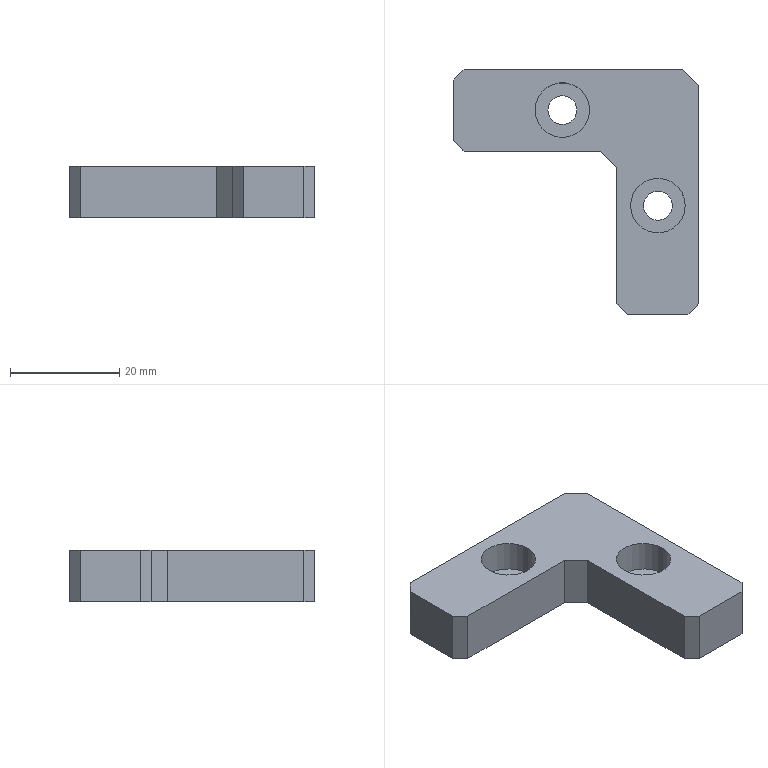Component | SolidWorks | --MA18S20041AxisStopBlock1-1 | 1 solid | 24 faces | box 45 x 45 x 9.5 mm | volume 9548 mm3 | plane 16 | cylinder 8 | commonest cylinder face diameters 10 x4 5.3 x4
build123d program:
from build123d import *

# Parameters (mm, degrees)
EXTRUDE_THIN1_DEPTH                                  = 9.5
CHAMFER1_SIZE                                        = 3
CHAMFER2_SIZE                                        = 2
HOLE_SIZE_ACCORDING_TO_THE_TYPE_OF_HEXAG_D           = 5.3
HOLE_SIZE_ACCORDING_TO_THE_TYPE_OF_HEXAG_CBORE_D     = 10
HOLE_SIZE_ACCORDING_TO_THE_TYPE_OF_HEXAG_CBORE_DEPTH = 5.7


with BuildPart() as part:
    # Sketch1 → Extrude-Thin1 (new body)
    with BuildSketch(Plane.XY):
        Polygon((0, 0), (45, 0), (45, -45), (30, -45), (30, -15), (0, -15), align=None)
    extrude(amount=EXTRUDE_THIN1_DEPTH)

    # Chamfer1
    chamfer1_edges = [part.edges().sort_by_distance(p)[0] for p in [
        (30, -15, 4.75),
        (45, 0, 4.75),
    ]]
    chamfer(chamfer1_edges, length=CHAMFER1_SIZE)

    # Chamfer2
    chamfer2_edges = [part.edges().sort_by_distance(p)[0] for p in [
        (0, -15, 4.75),
        (0, 0, 4.75),
        (45, -45, 4.75),
        (30, -45, 4.75),
    ]]
    chamfer(chamfer2_edges, length=CHAMFER2_SIZE)

    # Hole Size according to the type of Hexag (through all)
    with Locations(Plane.XY.offset(9.5)):
        with Locations((37.5, -25), (20, -7.5)):
            CounterBoreHole(HOLE_SIZE_ACCORDING_TO_THE_TYPE_OF_HEXAG_D / 2, HOLE_SIZE_ACCORDING_TO_THE_TYPE_OF_HEXAG_CBORE_D / 2, HOLE_SIZE_ACCORDING_TO_THE_TYPE_OF_HEXAG_CBORE_DEPTH)


solid = part.part

# Placed as in the assembly
solid = solid.moved(Location((-175.456, 104.199, 68), (0, 0, 0)))
STEP:
#1=COLOUR_RGB('',0.7922,0.8196,0.9333);
#2=FILL_AREA_STYLE_COLOUR('',#1);
#3=FILL_AREA_STYLE('',(#2));
#4=SURFACE_STYLE_FILL_AREA(#3);
#5=SURFACE_SIDE_STYLE('',(#4));
#6=SURFACE_STYLE_USAGE(.BOTH.,#5);
#7=PRESENTATION_STYLE_ASSIGNMENT((#6));
#8=CARTESIAN_POINT('',(-5.628,3.118,2.827));
#9=VERTEX_POINT('',#8);
#10=CARTESIAN_POINT('',(-5.234,3.118,2.827));
#11=VERTEX_POINT('',#10);
#12=CARTESIAN_POINT('',(-5.431,3.118,2.827));
#13=DIRECTION('',(0.,0.,1.));
#14=DIRECTION('',(1.,0.,0.));
#15=AXIS2_PLACEMENT_3D('',#12,#13,#14);
#16=CIRCLE('',#15,0.1969);
#17=EDGE_CURVE('',#9,#11,#16,.T.);
#18=ORIENTED_EDGE('',*,*,#17,.F.);
#19=CARTESIAN_POINT('',(-5.628,3.118,3.051));
#20=VERTEX_POINT('',#19);
#21=CARTESIAN_POINT('',(-5.628,3.118,3.051));
#22=DIRECTION('',(0.,0.,1.));
#23=VECTOR('',#22,39.37);
#24=LINE('',#21,#23);
#25=EDGE_CURVE('',#9,#20,#24,.T.);
#26=ORIENTED_EDGE('',*,*,#25,.T.);
#27=CARTESIAN_POINT('',(-5.234,3.118,3.051));
#28=VERTEX_POINT('',#27);
#29=CARTESIAN_POINT('',(-5.431,3.118,3.051));
#30=DIRECTION('',(0.,0.,1.));
#31=DIRECTION('',(1.,0.,0.));
#32=AXIS2_PLACEMENT_3D('',#29,#30,#31);
#33=CIRCLE('',#32,0.1969);
#34=EDGE_CURVE('',#20,#28,#33,.T.);
#35=ORIENTED_EDGE('',*,*,#34,.T.);
#36=CARTESIAN_POINT('',(-5.234,3.118,3.051));
#37=DIRECTION('',(0.,0.,1.));
#38=VECTOR('',#37,39.37);
#39=LINE('',#36,#38);
#40=EDGE_CURVE('',#11,#28,#39,.T.);
#41=ORIENTED_EDGE('',*,*,#40,.F.);
#42=EDGE_LOOP('',(#18,#26,#35,#41));
#43=FACE_OUTER_BOUND('',#42,.T.);
#44=CARTESIAN_POINT('',(-5.431,3.118,3.051));
#45=DIRECTION('',(0.,0.,1.));
#46=DIRECTION('',(1.,0.,0.));
#47=AXIS2_PLACEMENT_3D('',#44,#45,#46);
#48=CYLINDRICAL_SURFACE('',#47,0.1969);
#49=ADVANCED_FACE('',(#43),#48,.F.);
#50=CARTESIAN_POINT('',(-5.536,3.118,2.677));
#51=VERTEX_POINT('',#50);
#52=CARTESIAN_POINT('',(-5.327,3.118,2.677));
#53=VERTEX_POINT('',#52);
#54=CARTESIAN_POINT('',(-5.431,3.118,2.677));
#55=DIRECTION('',(0.,0.,1.));
#56=DIRECTION('',(1.,0.,0.));
#57=AXIS2_PLACEMENT_3D('',#54,#55,#56);
#58=CIRCLE('',#57,0.1043);
#59=EDGE_CURVE('',#51,#53,#58,.T.);
#60=ORIENTED_EDGE('',*,*,#59,.F.);
#61=CARTESIAN_POINT('',(-5.536,3.118,2.827));
#62=VERTEX_POINT('',#61);
#63=CARTESIAN_POINT('',(-5.536,3.118,3.051));
#64=DIRECTION('',(0.,0.,1.));
#65=VECTOR('',#64,39.37);
#66=LINE('',#63,#65);
#67=EDGE_CURVE('',#51,#62,#66,.T.);
#68=ORIENTED_EDGE('',*,*,#67,.T.);
#69=CARTESIAN_POINT('',(-5.327,3.118,2.827));
#70=VERTEX_POINT('',#69);
#71=CARTESIAN_POINT('',(-5.431,3.118,2.827));
#72=DIRECTION('',(0.,0.,1.));
#73=DIRECTION('',(1.,0.,0.));
#74=AXIS2_PLACEMENT_3D('',#71,#72,#73);
#75=CIRCLE('',#74,0.1043);
#76=EDGE_CURVE('',#62,#70,#75,.T.);
#77=ORIENTED_EDGE('',*,*,#76,.T.);
#78=CARTESIAN_POINT('',(-5.327,3.118,3.051));
#79=DIRECTION('',(0.,0.,1.));
#80=VECTOR('',#79,39.37);
#81=LINE('',#78,#80);
#82=EDGE_CURVE('',#53,#70,#81,.T.);
#83=ORIENTED_EDGE('',*,*,#82,.F.);
#84=EDGE_LOOP('',(#60,#68,#77,#83));
#85=FACE_OUTER_BOUND('',#84,.T.);
#86=CARTESIAN_POINT('',(-5.431,3.118,3.051));
#87=DIRECTION('',(0.,0.,1.));
#88=DIRECTION('',(1.,0.,0.));
#89=AXIS2_PLACEMENT_3D('',#86,#87,#88);
#90=CYLINDRICAL_SURFACE('',#89,0.1043);
#91=ADVANCED_FACE('',(#85),#90,.F.);
#92=CARTESIAN_POINT('',(-6.317,3.807,2.827));
#93=VERTEX_POINT('',#92);
#94=CARTESIAN_POINT('',(-5.923,3.807,2.827));
#95=VERTEX_POINT('',#94);
#96=CARTESIAN_POINT('',(-6.12,3.807,2.827));
#97=DIRECTION('',(0.,0.,1.));
#98=DIRECTION('',(1.,0.,0.));
#99=AXIS2_PLACEMENT_3D('',#96,#97,#98);
#100=CIRCLE('',#99,0.1969);
#101=EDGE_CURVE('',#93,#95,#100,.T.);
#102=ORIENTED_EDGE('',*,*,#101,.F.);
#103=CARTESIAN_POINT('',(-6.317,3.807,3.051));
#104=VERTEX_POINT('',#103);
#105=CARTESIAN_POINT('',(-6.317,3.807,3.051));
#106=DIRECTION('',(0.,0.,1.));
#107=VECTOR('',#106,39.37);
#108=LINE('',#105,#107);
#109=EDGE_CURVE('',#93,#104,#108,.T.);
#110=ORIENTED_EDGE('',*,*,#109,.T.);
#111=CARTESIAN_POINT('',(-5.923,3.807,3.051));
#112=VERTEX_POINT('',#111);
#113=CARTESIAN_POINT('',(-6.12,3.807,3.051));
#114=DIRECTION('',(0.,0.,1.));
#115=DIRECTION('',(1.,0.,0.));
#116=AXIS2_PLACEMENT_3D('',#113,#114,#115);
#117=CIRCLE('',#116,0.1969);
#118=EDGE_CURVE('',#104,#112,#117,.T.);
#119=ORIENTED_EDGE('',*,*,#118,.T.);
#120=CARTESIAN_POINT('',(-5.923,3.807,3.051));
#121=DIRECTION('',(0.,0.,1.));
#122=VECTOR('',#121,39.37);
#123=LINE('',#120,#122);
#124=EDGE_CURVE('',#95,#112,#123,.T.);
#125=ORIENTED_EDGE('',*,*,#124,.F.);
#126=EDGE_LOOP('',(#102,#110,#119,#125));
#127=FACE_OUTER_BOUND('',#126,.T.);
#128=CARTESIAN_POINT('',(-6.12,3.807,3.051));
#129=DIRECTION('',(0.,0.,1.));
#130=DIRECTION('',(1.,0.,0.));
#131=AXIS2_PLACEMENT_3D('',#128,#129,#130);
#132=CYLINDRICAL_SURFACE('',#131,0.1969);
#133=ADVANCED_FACE('',(#127),#132,.F.);
#134=CARTESIAN_POINT('',(-6.225,3.807,2.677));
#135=VERTEX_POINT('',#134);
#136=CARTESIAN_POINT('',(-6.016,3.807,2.677));
#137=VERTEX_POINT('',#136);
#138=CARTESIAN_POINT('',(-6.12,3.807,2.677));
#139=DIRECTION('',(0.,0.,1.));
#140=DIRECTION('',(1.,0.,0.));
#141=AXIS2_PLACEMENT_3D('',#138,#139,#140);
#142=CIRCLE('',#141,0.1043);
#143=EDGE_CURVE('',#135,#137,#142,.T.);
#144=ORIENTED_EDGE('',*,*,#143,.F.);
#145=CARTESIAN_POINT('',(-6.225,3.807,2.827));
#146=VERTEX_POINT('',#145);
#147=CARTESIAN_POINT('',(-6.225,3.807,3.051));
#148=DIRECTION('',(0.,0.,1.));
#149=VECTOR('',#148,39.37);
#150=LINE('',#147,#149);
#151=EDGE_CURVE('',#135,#146,#150,.T.);
#152=ORIENTED_EDGE('',*,*,#151,.T.);
#153=CARTESIAN_POINT('',(-6.016,3.807,2.827));
#154=VERTEX_POINT('',#153);
#155=CARTESIAN_POINT('',(-6.12,3.807,2.827));
#156=DIRECTION('',(0.,0.,1.));
#157=DIRECTION('',(1.,0.,0.));
#158=AXIS2_PLACEMENT_3D('',#155,#156,#157);
#159=CIRCLE('',#158,0.1043);
#160=EDGE_CURVE('',#146,#154,#159,.T.);
#161=ORIENTED_EDGE('',*,*,#160,.T.);
#162=CARTESIAN_POINT('',(-6.016,3.807,3.051));
#163=DIRECTION('',(0.,0.,1.));
#164=VECTOR('',#163,39.37);
#165=LINE('',#162,#164);
#166=EDGE_CURVE('',#137,#154,#165,.T.);
#167=ORIENTED_EDGE('',*,*,#166,.F.);
#168=EDGE_LOOP('',(#144,#152,#161,#167));
#169=FACE_OUTER_BOUND('',#168,.T.);
#170=CARTESIAN_POINT('',(-6.12,3.807,3.051));
#171=DIRECTION('',(0.,0.,1.));
#172=DIRECTION('',(1.,0.,0.));
#173=AXIS2_PLACEMENT_3D('',#170,#171,#172);
#174=CYLINDRICAL_SURFACE('',#173,0.1043);
#175=ADVANCED_FACE('',(#169),#174,.F.);
#176=CARTESIAN_POINT('',(-5.431,3.118,3.051));
#177=DIRECTION('',(0.,0.,1.));
#178=DIRECTION('',(1.,0.,0.));
#179=AXIS2_PLACEMENT_3D('',#176,#177,#178);
#180=CIRCLE('',#179,0.1969);
#181=EDGE_CURVE('',#28,#20,#180,.T.);
#182=ORIENTED_EDGE('',*,*,#181,.F.);
#183=ORIENTED_EDGE('',*,*,#34,.F.);
#184=EDGE_LOOP('',(#182,#183));
#185=FACE_BOUND('',#184,.T.);
#186=CARTESIAN_POINT('',(-5.215,2.331,3.051));
#187=VERTEX_POINT('',#186);
#188=CARTESIAN_POINT('',(-5.648,2.331,3.051));
#189=VERTEX_POINT('',#188);
#190=CARTESIAN_POINT('',(-5.136,2.331,3.051));
#191=DIRECTION('',(-1.,0.,0.));
#192=VECTOR('',#191,39.37);
#193=LINE('',#190,#192);
#194=EDGE_CURVE('',#187,#189,#193,.T.);
#195=ORIENTED_EDGE('',*,*,#194,.F.);
#196=CARTESIAN_POINT('',(-5.136,2.409,3.051));
#197=VERTEX_POINT('',#196);
#198=CARTESIAN_POINT('',(-5.136,2.409,3.051));
#199=DIRECTION('',(0.7071,0.7071,0.));
#200=VECTOR('',#199,39.37);
#201=LINE('',#198,#200);
#202=EDGE_CURVE('',#187,#197,#201,.T.);
#203=ORIENTED_EDGE('',*,*,#202,.T.);
#204=CARTESIAN_POINT('',(-5.136,3.984,3.051));
#205=VERTEX_POINT('',#204);
#206=CARTESIAN_POINT('',(-5.136,4.102,3.051));
#207=DIRECTION('',(0.,-1.,0.));
#208=VECTOR('',#207,39.37);
#209=LINE('',#206,#208);
#210=EDGE_CURVE('',#205,#197,#209,.T.);
#211=ORIENTED_EDGE('',*,*,#210,.F.);
#212=CARTESIAN_POINT('',(-5.254,4.102,3.051));
#213=VERTEX_POINT('',#212);
#214=CARTESIAN_POINT('',(-5.254,4.102,3.051));
#215=DIRECTION('',(-0.7071,0.7071,0.));
#216=VECTOR('',#215,39.37);
#217=LINE('',#214,#216);
#218=EDGE_CURVE('',#205,#213,#217,.T.);
#219=ORIENTED_EDGE('',*,*,#218,.T.);
#220=CARTESIAN_POINT('',(-6.829,4.102,3.051));
#221=VERTEX_POINT('',#220);
#222=CARTESIAN_POINT('',(-6.908,4.102,3.051));
#223=DIRECTION('',(1.,0.,0.));
#224=VECTOR('',#223,39.37);
#225=LINE('',#222,#224);
#226=EDGE_CURVE('',#221,#213,#225,.T.);
#227=ORIENTED_EDGE('',*,*,#226,.F.);
#228=CARTESIAN_POINT('',(-6.908,4.024,3.051));
#229=VERTEX_POINT('',#228);
#230=CARTESIAN_POINT('',(-6.908,4.024,3.051));
#231=DIRECTION('',(-0.7071,-0.7071,0.));
#232=VECTOR('',#231,39.37);
#233=LINE('',#230,#232);
#234=EDGE_CURVE('',#221,#229,#233,.T.);
#235=ORIENTED_EDGE('',*,*,#234,.T.);
#236=CARTESIAN_POINT('',(-6.908,3.591,3.051));
#237=VERTEX_POINT('',#236);
#238=CARTESIAN_POINT('',(-6.908,3.512,3.051));
#239=DIRECTION('',(0.,1.,0.));
#240=VECTOR('',#239,39.37);
#241=LINE('',#238,#240);
#242=EDGE_CURVE('',#237,#229,#241,.T.);
#243=ORIENTED_EDGE('',*,*,#242,.F.);
#244=CARTESIAN_POINT('',(-6.829,3.512,3.051));
#245=VERTEX_POINT('',#244);
#246=CARTESIAN_POINT('',(-6.829,3.512,3.051));
#247=DIRECTION('',(0.7071,-0.7071,0.));
#248=VECTOR('',#247,39.37);
#249=LINE('',#246,#248);
#250=EDGE_CURVE('',#237,#245,#249,.T.);
#251=ORIENTED_EDGE('',*,*,#250,.T.);
#252=CARTESIAN_POINT('',(-5.845,3.512,3.051));
#253=VERTEX_POINT('',#252);
#254=CARTESIAN_POINT('',(-6.908,3.512,3.051));
#255=DIRECTION('',(1.,0.,0.));
#256=VECTOR('',#255,39.37);
#257=LINE('',#254,#256);
#258=EDGE_CURVE('',#245,#253,#257,.T.);
#259=ORIENTED_EDGE('',*,*,#258,.T.);
#260=CARTESIAN_POINT('',(-5.727,3.394,3.051));
#261=VERTEX_POINT('',#260);
#262=CARTESIAN_POINT('',(-5.195,2.862,3.051));
#263=DIRECTION('',(0.7071,-0.7071,0.));
#264=VECTOR('',#263,39.37);
#265=LINE('',#262,#264);
#266=EDGE_CURVE('',#253,#261,#265,.T.);
#267=ORIENTED_EDGE('',*,*,#266,.T.);
#268=CARTESIAN_POINT('',(-5.727,2.409,3.051));
#269=VERTEX_POINT('',#268);
#270=CARTESIAN_POINT('',(-5.727,4.102,3.051));
#271=DIRECTION('',(0.,-1.,0.));
#272=VECTOR('',#271,39.37);
#273=LINE('',#270,#272);
#274=EDGE_CURVE('',#261,#269,#273,.T.);
#275=ORIENTED_EDGE('',*,*,#274,.T.);
#276=CARTESIAN_POINT('',(-5.648,2.331,3.051));
#277=DIRECTION('',(0.7071,-0.7071,0.));
#278=VECTOR('',#277,39.37);
#279=LINE('',#276,#278);
#280=EDGE_CURVE('',#269,#189,#279,.T.);
#281=ORIENTED_EDGE('',*,*,#280,.T.);
#282=EDGE_LOOP('',(#195,#203,#211,#219,#227,#235,#243,#251,#259,#267,#275,#281));
#283=FACE_OUTER_BOUND('',#282,.T.);
#284=CARTESIAN_POINT('',(-6.12,3.807,3.051));
#285=DIRECTION('',(0.,0.,1.));
#286=DIRECTION('',(1.,0.,0.));
#287=AXIS2_PLACEMENT_3D('',#284,#285,#286);
#288=CIRCLE('',#287,0.1969);
#289=EDGE_CURVE('',#112,#104,#288,.T.);
#290=ORIENTED_EDGE('',*,*,#289,.F.);
#291=ORIENTED_EDGE('',*,*,#118,.F.);
#292=EDGE_LOOP('',(#290,#291));
#293=FACE_BOUND('',#292,.T.);
#294=CARTESIAN_POINT('',(-5.727,2.331,3.051));
#295=DIRECTION('',(0.,0.,-1.));
#296=DIRECTION('',(-1.,0.,0.));
#297=AXIS2_PLACEMENT_3D('',#294,#295,#296);
#298=PLANE('',#297);
#299=ADVANCED_FACE('',(#185,#283,#293),#298,.F.);
#300=CARTESIAN_POINT('',(-5.727,3.394,2.677));
#301=VERTEX_POINT('',#300);
#302=CARTESIAN_POINT('',(-5.727,2.409,2.677));
#303=VERTEX_POINT('',#302);
#304=CARTESIAN_POINT('',(-5.727,4.102,2.677));
#305=DIRECTION('',(0.,-1.,0.));
#306=VECTOR('',#305,39.37);
#307=LINE('',#304,#306);
#308=EDGE_CURVE('',#301,#303,#307,.T.);
#309=ORIENTED_EDGE('',*,*,#308,.T.);
#310=CARTESIAN_POINT('',(-5.727,2.409,3.051));
#311=DIRECTION('',(0.,0.,1.));
#312=VECTOR('',#311,39.37);
#313=LINE('',#310,#312);
#314=EDGE_CURVE('',#303,#269,#313,.T.);
#315=ORIENTED_EDGE('',*,*,#314,.T.);
#316=ORIENTED_EDGE('',*,*,#274,.F.);
#317=CARTESIAN_POINT('',(-5.727,3.394,2.677));
#318=DIRECTION('',(0.,0.,-1.));
#319=VECTOR('',#318,39.37);
#320=LINE('',#317,#319);
#321=EDGE_CURVE('',#261,#301,#320,.T.);
#322=ORIENTED_EDGE('',*,*,#321,.T.);
#323=EDGE_LOOP('',(#309,#315,#316,#322));
#324=FACE_OUTER_BOUND('',#323,.T.);
#325=CARTESIAN_POINT('',(-5.727,4.102,3.051));
#326=DIRECTION('',(1.,0.,0.));
#327=DIRECTION('',(-0.,1.,0.));
#328=AXIS2_PLACEMENT_3D('',#325,#326,#327);
#329=PLANE('',#328);
#330=ADVANCED_FACE('',(#324),#329,.F.);
#331=CARTESIAN_POINT('',(-5.215,2.331,2.677));
#332=VERTEX_POINT('',#331);
#333=CARTESIAN_POINT('',(-5.648,2.331,2.677));
#334=VERTEX_POINT('',#333);
#335=CARTESIAN_POINT('',(-5.136,2.331,2.677));
#336=DIRECTION('',(-1.,0.,0.));
#337=VECTOR('',#336,39.37);
#338=LINE('',#335,#337);
#339=EDGE_CURVE('',#332,#334,#338,.T.);
#340=ORIENTED_EDGE('',*,*,#339,.F.);
#341=CARTESIAN_POINT('',(-5.215,2.331,3.051));
#342=DIRECTION('',(0.,0.,1.));
#343=VECTOR('',#342,39.37);
#344=LINE('',#341,#343);
#345=EDGE_CURVE('',#332,#187,#344,.T.);
#346=ORIENTED_EDGE('',*,*,#345,.T.);
#347=ORIENTED_EDGE('',*,*,#194,.T.);
#348=CARTESIAN_POINT('',(-5.648,2.331,2.677));
#349=DIRECTION('',(0.,0.,-1.));
#350=VECTOR('',#349,39.37);
#351=LINE('',#348,#350);
#352=EDGE_CURVE('',#189,#334,#351,.T.);
#353=ORIENTED_EDGE('',*,*,#352,.T.);
#354=EDGE_LOOP('',(#340,#346,#347,#353));
#355=FACE_OUTER_BOUND('',#354,.T.);
#356=CARTESIAN_POINT('',(-5.136,2.331,3.051));
#357=DIRECTION('',(0.,-1.,0.));
#358=DIRECTION('',(0.,0.,-1.));
#359=AXIS2_PLACEMENT_3D('',#356,#357,#358);
#360=PLANE('',#359);
#361=ADVANCED_FACE('',(#355),#360,.T.);
#362=ORIENTED_EDGE('',*,*,#210,.T.);
#363=CARTESIAN_POINT('',(-5.136,2.409,2.677));
#364=VERTEX_POINT('',#363);
#365=CARTESIAN_POINT('',(-5.136,2.409,3.051));
#366=DIRECTION('',(0.,0.,-1.));
#367=VECTOR('',#366,39.37);
#368=LINE('',#365,#367);
#369=EDGE_CURVE('',#197,#364,#368,.T.);
#370=ORIENTED_EDGE('',*,*,#369,.T.);
#371=CARTESIAN_POINT('',(-5.136,3.984,2.677));
#372=VERTEX_POINT('',#371);
#373=CARTESIAN_POINT('',(-5.136,4.102,2.677));
#374=DIRECTION('',(0.,-1.,0.));
#375=VECTOR('',#374,39.37);
#376=LINE('',#373,#375);
#377=EDGE_CURVE('',#372,#364,#376,.T.);
#378=ORIENTED_EDGE('',*,*,#377,.F.);
#379=CARTESIAN_POINT('',(-5.136,3.984,3.051));
#380=DIRECTION('',(0.,0.,1.));
#381=VECTOR('',#380,39.37);
#382=LINE('',#379,#381);
#383=EDGE_CURVE('',#372,#205,#382,.T.);
#384=ORIENTED_EDGE('',*,*,#383,.T.);
#385=EDGE_LOOP('',(#362,#370,#378,#384));
#386=FACE_OUTER_BOUND('',#385,.T.);
#387=CARTESIAN_POINT('',(-5.136,4.102,3.051));
#388=DIRECTION('',(1.,0.,0.));
#389=DIRECTION('',(-0.,1.,0.));
#390=AXIS2_PLACEMENT_3D('',#387,#388,#389);
#391=PLANE('',#390);
#392=ADVANCED_FACE('',(#386),#391,.T.);
#393=CARTESIAN_POINT('',(-6.829,4.102,2.677));
#394=VERTEX_POINT('',#393);
#395=CARTESIAN_POINT('',(-5.254,4.102,2.677));
#396=VERTEX_POINT('',#395);
#397=CARTESIAN_POINT('',(-6.908,4.102,2.677));
#398=DIRECTION('',(1.,0.,0.));
#399=VECTOR('',#398,39.37);
#400=LINE('',#397,#399);
#401=EDGE_CURVE('',#394,#396,#400,.T.);
#402=ORIENTED_EDGE('',*,*,#401,.F.);
#403=CARTESIAN_POINT('',(-6.829,4.102,3.051));
#404=DIRECTION('',(0.,0.,1.));
#405=VECTOR('',#404,39.37);
#406=LINE('',#403,#405);
#407=EDGE_CURVE('',#394,#221,#406,.T.);
#408=ORIENTED_EDGE('',*,*,#407,.T.);
#409=ORIENTED_EDGE('',*,*,#226,.T.);
#410=CARTESIAN_POINT('',(-5.254,4.102,3.051));
#411=DIRECTION('',(0.,0.,-1.));
#412=VECTOR('',#411,39.37);
#413=LINE('',#410,#412);
#414=EDGE_CURVE('',#213,#396,#413,.T.);
#415=ORIENTED_EDGE('',*,*,#414,.T.);
#416=EDGE_LOOP('',(#402,#408,#409,#415));
#417=FACE_OUTER_BOUND('',#416,.T.);
#418=CARTESIAN_POINT('',(-6.908,4.102,3.051));
#419=DIRECTION('',(0.,1.,0.));
#420=DIRECTION('',(0.,0.,1.));
#421=AXIS2_PLACEMENT_3D('',#418,#419,#420);
#422=PLANE('',#421);
#423=ADVANCED_FACE('',(#417),#422,.T.);
#424=CARTESIAN_POINT('',(-6.908,3.591,2.677));
#425=VERTEX_POINT('',#424);
#426=CARTESIAN_POINT('',(-6.908,4.024,2.677));
#427=VERTEX_POINT('',#426);
#428=CARTESIAN_POINT('',(-6.908,3.512,2.677));
#429=DIRECTION('',(0.,1.,0.));
#430=VECTOR('',#429,39.37);
#431=LINE('',#428,#430);
#432=EDGE_CURVE('',#425,#427,#431,.T.);
#433=ORIENTED_EDGE('',*,*,#432,.F.);
#434=CARTESIAN_POINT('',(-6.908,3.591,3.051));
#435=DIRECTION('',(0.,0.,1.));
#436=VECTOR('',#435,39.37);
#437=LINE('',#434,#436);
#438=EDGE_CURVE('',#425,#237,#437,.T.);
#439=ORIENTED_EDGE('',*,*,#438,.T.);
#440=ORIENTED_EDGE('',*,*,#242,.T.);
#441=CARTESIAN_POINT('',(-6.908,4.024,3.051));
#442=DIRECTION('',(0.,0.,-1.));
#443=VECTOR('',#442,39.37);
#444=LINE('',#441,#443);
#445=EDGE_CURVE('',#229,#427,#444,.T.);
#446=ORIENTED_EDGE('',*,*,#445,.T.);
#447=EDGE_LOOP('',(#433,#439,#440,#446));
#448=FACE_OUTER_BOUND('',#447,.T.);
#449=CARTESIAN_POINT('',(-6.908,3.512,3.051));
#450=DIRECTION('',(-1.,0.,0.));
#451=DIRECTION('',(0.,0.,1.));
#452=AXIS2_PLACEMENT_3D('',#449,#450,#451);
#453=PLANE('',#452);
#454=ADVANCED_FACE('',(#448),#453,.T.);
#455=ORIENTED_EDGE('',*,*,#258,.F.);
#456=CARTESIAN_POINT('',(-6.829,3.512,2.677));
#457=VERTEX_POINT('',#456);
#458=CARTESIAN_POINT('',(-6.829,3.512,2.677));
#459=DIRECTION('',(0.,0.,-1.));
#460=VECTOR('',#459,39.37);
#461=LINE('',#458,#460);
#462=EDGE_CURVE('',#245,#457,#461,.T.);
#463=ORIENTED_EDGE('',*,*,#462,.T.);
#464=CARTESIAN_POINT('',(-5.845,3.512,2.677));
#465=VERTEX_POINT('',#464);
#466=CARTESIAN_POINT('',(-6.908,3.512,2.677));
#467=DIRECTION('',(1.,0.,0.));
#468=VECTOR('',#467,39.37);
#469=LINE('',#466,#468);
#470=EDGE_CURVE('',#457,#465,#469,.T.);
#471=ORIENTED_EDGE('',*,*,#470,.T.);
#472=CARTESIAN_POINT('',(-5.845,3.512,3.051));
#473=DIRECTION('',(0.,0.,1.));
#474=VECTOR('',#473,39.37);
#475=LINE('',#472,#474);
#476=EDGE_CURVE('',#465,#253,#475,.T.);
#477=ORIENTED_EDGE('',*,*,#476,.T.);
#478=EDGE_LOOP('',(#455,#463,#471,#477));
#479=FACE_OUTER_BOUND('',#478,.T.);
#480=CARTESIAN_POINT('',(-6.908,3.512,3.051));
#481=DIRECTION('',(0.,1.,0.));
#482=DIRECTION('',(0.,0.,1.));
#483=AXIS2_PLACEMENT_3D('',#480,#481,#482);
#484=PLANE('',#483);
#485=ADVANCED_FACE('',(#479),#484,.F.);
#486=CARTESIAN_POINT('',(-5.431,3.118,2.677));
#487=DIRECTION('',(0.,0.,1.));
#488=DIRECTION('',(1.,0.,0.));
#489=AXIS2_PLACEMENT_3D('',#486,#487,#488);
#490=CIRCLE('',#489,0.1043);
#491=EDGE_CURVE('',#53,#51,#490,.T.);
#492=ORIENTED_EDGE('',*,*,#491,.T.);
#493=ORIENTED_EDGE('',*,*,#59,.T.);
#494=EDGE_LOOP('',(#492,#493));
#495=FACE_BOUND('',#494,.T.);
#496=CARTESIAN_POINT('',(-6.12,3.807,2.677));
#497=DIRECTION('',(0.,0.,1.));
#498=DIRECTION('',(1.,0.,0.));
#499=AXIS2_PLACEMENT_3D('',#496,#497,#498);
#500=CIRCLE('',#499,0.1043);
#501=EDGE_CURVE('',#137,#135,#500,.T.);
#502=ORIENTED_EDGE('',*,*,#501,.T.);
#503=ORIENTED_EDGE('',*,*,#143,.T.);
#504=EDGE_LOOP('',(#502,#503));
#505=FACE_BOUND('',#504,.T.);
#506=ORIENTED_EDGE('',*,*,#377,.T.);
#507=CARTESIAN_POINT('',(-5.471,2.075,2.677));
#508=DIRECTION('',(-0.7071,-0.7071,0.));
#509=VECTOR('',#508,39.37);
#510=LINE('',#507,#509);
#511=EDGE_CURVE('',#364,#332,#510,.T.);
#512=ORIENTED_EDGE('',*,*,#511,.T.);
#513=ORIENTED_EDGE('',*,*,#339,.T.);
#514=CARTESIAN_POINT('',(-5.687,2.37,2.677));
#515=DIRECTION('',(-0.7071,0.7071,0.));
#516=VECTOR('',#515,39.37);
#517=LINE('',#514,#516);
#518=EDGE_CURVE('',#334,#303,#517,.T.);
#519=ORIENTED_EDGE('',*,*,#518,.T.);
#520=ORIENTED_EDGE('',*,*,#308,.F.);
#521=CARTESIAN_POINT('',(-5.727,3.394,2.677));
#522=DIRECTION('',(-0.7071,0.7071,0.));
#523=VECTOR('',#522,39.37);
#524=LINE('',#521,#523);
#525=EDGE_CURVE('',#301,#465,#524,.T.);
#526=ORIENTED_EDGE('',*,*,#525,.T.);
#527=ORIENTED_EDGE('',*,*,#470,.F.);
#528=CARTESIAN_POINT('',(-5.687,2.37,2.677));
#529=DIRECTION('',(-0.7071,0.7071,0.));
#530=VECTOR('',#529,39.37);
#531=LINE('',#528,#530);
#532=EDGE_CURVE('',#457,#425,#531,.T.);
#533=ORIENTED_EDGE('',*,*,#532,.T.);
#534=ORIENTED_EDGE('',*,*,#432,.T.);
#535=CARTESIAN_POINT('',(-7.164,3.768,2.677));
#536=DIRECTION('',(0.7071,0.7071,0.));
#537=VECTOR('',#536,39.37);
#538=LINE('',#535,#537);
#539=EDGE_CURVE('',#427,#394,#538,.T.);
#540=ORIENTED_EDGE('',*,*,#539,.T.);
#541=ORIENTED_EDGE('',*,*,#401,.T.);
#542=CARTESIAN_POINT('',(-4.605,3.453,2.677));
#543=DIRECTION('',(0.7071,-0.7071,0.));
#544=VECTOR('',#543,39.37);
#545=LINE('',#542,#544);
#546=EDGE_CURVE('',#396,#372,#545,.T.);
#547=ORIENTED_EDGE('',*,*,#546,.T.);
#548=EDGE_LOOP('',(#506,#512,#513,#519,#520,#526,#527,#533,#534,#540,#541,#547));
#549=FACE_OUTER_BOUND('',#548,.T.);
#550=CARTESIAN_POINT('',(-5.727,2.331,2.677));
#551=DIRECTION('',(0.,0.,-1.));
#552=DIRECTION('',(-1.,0.,0.));
#553=AXIS2_PLACEMENT_3D('',#550,#551,#552);
#554=PLANE('',#553);
#555=ADVANCED_FACE('',(#495,#505,#549),#554,.T.);
#556=ORIENTED_EDGE('',*,*,#266,.F.);
#557=ORIENTED_EDGE('',*,*,#476,.F.);
#558=ORIENTED_EDGE('',*,*,#525,.F.);
#559=ORIENTED_EDGE('',*,*,#321,.F.);
#560=EDGE_LOOP('',(#556,#557,#558,#559));
#561=FACE_OUTER_BOUND('',#560,.T.);
#562=CARTESIAN_POINT('',(-5.727,3.394,3.051));
#563=DIRECTION('',(-0.7071,-0.7071,0.));
#564=DIRECTION('',(0.7071,-0.7071,0.));
#565=AXIS2_PLACEMENT_3D('',#562,#563,#564);
#566=PLANE('',#565);
#567=ADVANCED_FACE('',(#561),#566,.T.);
#568=ORIENTED_EDGE('',*,*,#218,.F.);
#569=ORIENTED_EDGE('',*,*,#383,.F.);
#570=ORIENTED_EDGE('',*,*,#546,.F.);
#571=ORIENTED_EDGE('',*,*,#414,.F.);
#572=EDGE_LOOP('',(#568,#569,#570,#571));
#573=FACE_OUTER_BOUND('',#572,.T.);
#574=CARTESIAN_POINT('',(-5.254,4.102,3.051));
#575=DIRECTION('',(-0.7071,-0.7071,0.));
#576=DIRECTION('',(0.7071,-0.7071,0.));
#577=AXIS2_PLACEMENT_3D('',#574,#575,#576);
#578=PLANE('',#577);
#579=ADVANCED_FACE('',(#573),#578,.F.);
#580=ORIENTED_EDGE('',*,*,#202,.F.);
#581=ORIENTED_EDGE('',*,*,#345,.F.);
#582=ORIENTED_EDGE('',*,*,#511,.F.);
#583=ORIENTED_EDGE('',*,*,#369,.F.);
#584=EDGE_LOOP('',(#580,#581,#582,#583));
#585=FACE_OUTER_BOUND('',#584,.T.);
#586=CARTESIAN_POINT('',(-5.136,2.409,3.051));
#587=DIRECTION('',(-0.7071,0.7071,0.));
#588=DIRECTION('',(-0.7071,-0.7071,0.));
#589=AXIS2_PLACEMENT_3D('',#586,#587,#588);
#590=PLANE('',#589);
#591=ADVANCED_FACE('',(#585),#590,.F.);
#592=ORIENTED_EDGE('',*,*,#280,.F.);
#593=ORIENTED_EDGE('',*,*,#314,.F.);
#594=ORIENTED_EDGE('',*,*,#518,.F.);
#595=ORIENTED_EDGE('',*,*,#352,.F.);
#596=EDGE_LOOP('',(#592,#593,#594,#595));
#597=FACE_OUTER_BOUND('',#596,.T.);
#598=CARTESIAN_POINT('',(-5.648,2.331,3.051));
#599=DIRECTION('',(-0.7071,-0.7071,0.));
#600=DIRECTION('',(0.7071,-0.7071,0.));
#601=AXIS2_PLACEMENT_3D('',#598,#599,#600);
#602=PLANE('',#601);
#603=ADVANCED_FACE('',(#597),#602,.T.);
#604=ORIENTED_EDGE('',*,*,#250,.F.);
#605=ORIENTED_EDGE('',*,*,#438,.F.);
#606=ORIENTED_EDGE('',*,*,#532,.F.);
#607=ORIENTED_EDGE('',*,*,#462,.F.);
#608=EDGE_LOOP('',(#604,#605,#606,#607));
#609=FACE_OUTER_BOUND('',#608,.T.);
#610=CARTESIAN_POINT('',(-6.829,3.512,3.051));
#611=DIRECTION('',(-0.7071,-0.7071,0.));
#612=DIRECTION('',(0.7071,-0.7071,0.));
#613=AXIS2_PLACEMENT_3D('',#610,#611,#612);
#614=PLANE('',#613);
#615=ADVANCED_FACE('',(#609),#614,.T.);
#616=ORIENTED_EDGE('',*,*,#234,.F.);
#617=ORIENTED_EDGE('',*,*,#407,.F.);
#618=ORIENTED_EDGE('',*,*,#539,.F.);
#619=ORIENTED_EDGE('',*,*,#445,.F.);
#620=EDGE_LOOP('',(#616,#617,#618,#619));
#621=FACE_OUTER_BOUND('',#620,.T.);
#622=CARTESIAN_POINT('',(-6.908,4.024,3.051));
#623=DIRECTION('',(0.7071,-0.7071,0.));
#624=DIRECTION('',(0.7071,0.7071,0.));
#625=AXIS2_PLACEMENT_3D('',#622,#623,#624);
#626=PLANE('',#625);
#627=ADVANCED_FACE('',(#621),#626,.F.);
#628=ORIENTED_EDGE('',*,*,#151,.F.);
#629=ORIENTED_EDGE('',*,*,#501,.F.);
#630=ORIENTED_EDGE('',*,*,#166,.T.);
#631=CARTESIAN_POINT('',(-6.12,3.807,2.827));
#632=DIRECTION('',(0.,0.,1.));
#633=DIRECTION('',(1.,0.,0.));
#634=AXIS2_PLACEMENT_3D('',#631,#632,#633);
#635=CIRCLE('',#634,0.1043);
#636=EDGE_CURVE('',#154,#146,#635,.T.);
#637=ORIENTED_EDGE('',*,*,#636,.T.);
#638=EDGE_LOOP('',(#628,#629,#630,#637));
#639=FACE_OUTER_BOUND('',#638,.T.);
#640=CARTESIAN_POINT('',(-6.12,3.807,3.051));
#641=DIRECTION('',(0.,0.,1.));
#642=DIRECTION('',(1.,0.,0.));
#643=AXIS2_PLACEMENT_3D('',#640,#641,#642);
#644=CYLINDRICAL_SURFACE('',#643,0.1043);
#645=ADVANCED_FACE('',(#639),#644,.F.);
#646=ORIENTED_EDGE('',*,*,#636,.F.);
#647=ORIENTED_EDGE('',*,*,#160,.F.);
#648=EDGE_LOOP('',(#646,#647));
#649=FACE_BOUND('',#648,.T.);
#650=CARTESIAN_POINT('',(-6.12,3.807,2.827));
#651=DIRECTION('',(0.,0.,1.));
#652=DIRECTION('',(1.,0.,0.));
#653=AXIS2_PLACEMENT_3D('',#650,#651,#652);
#654=CIRCLE('',#653,0.1969);
#655=EDGE_CURVE('',#95,#93,#654,.T.);
#656=ORIENTED_EDGE('',*,*,#655,.T.);
#657=ORIENTED_EDGE('',*,*,#101,.T.);
#658=EDGE_LOOP('',(#656,#657));
#659=FACE_OUTER_BOUND('',#658,.T.);
#660=CARTESIAN_POINT('',(-6.016,3.807,2.827));
#661=DIRECTION('',(0.,0.,-1.));
#662=DIRECTION('',(-1.,0.,0.));
#663=AXIS2_PLACEMENT_3D('',#660,#661,#662);
#664=PLANE('',#663);
#665=ADVANCED_FACE('',(#649,#659),#664,.F.);
#666=ORIENTED_EDGE('',*,*,#109,.F.);
#667=ORIENTED_EDGE('',*,*,#655,.F.);
#668=ORIENTED_EDGE('',*,*,#124,.T.);
#669=ORIENTED_EDGE('',*,*,#289,.T.);
#670=EDGE_LOOP('',(#666,#667,#668,#669));
#671=FACE_OUTER_BOUND('',#670,.T.);
#672=CARTESIAN_POINT('',(-6.12,3.807,3.051));
#673=DIRECTION('',(0.,0.,1.));
#674=DIRECTION('',(1.,0.,0.));
#675=AXIS2_PLACEMENT_3D('',#672,#673,#674);
#676=CYLINDRICAL_SURFACE('',#675,0.1969);
#677=ADVANCED_FACE('',(#671),#676,.F.);
#678=ORIENTED_EDGE('',*,*,#67,.F.);
#679=ORIENTED_EDGE('',*,*,#491,.F.);
#680=ORIENTED_EDGE('',*,*,#82,.T.);
#681=CARTESIAN_POINT('',(-5.431,3.118,2.827));
#682=DIRECTION('',(0.,0.,1.));
#683=DIRECTION('',(1.,0.,0.));
#684=AXIS2_PLACEMENT_3D('',#681,#682,#683);
#685=CIRCLE('',#684,0.1043);
#686=EDGE_CURVE('',#70,#62,#685,.T.);
#687=ORIENTED_EDGE('',*,*,#686,.T.);
#688=EDGE_LOOP('',(#678,#679,#680,#687));
#689=FACE_OUTER_BOUND('',#688,.T.);
#690=CARTESIAN_POINT('',(-5.431,3.118,3.051));
#691=DIRECTION('',(0.,0.,1.));
#692=DIRECTION('',(1.,0.,0.));
#693=AXIS2_PLACEMENT_3D('',#690,#691,#692);
#694=CYLINDRICAL_SURFACE('',#693,0.1043);
#695=ADVANCED_FACE('',(#689),#694,.F.);
#696=ORIENTED_EDGE('',*,*,#686,.F.);
#697=ORIENTED_EDGE('',*,*,#76,.F.);
#698=EDGE_LOOP('',(#696,#697));
#699=FACE_BOUND('',#698,.T.);
#700=CARTESIAN_POINT('',(-5.431,3.118,2.827));
#701=DIRECTION('',(0.,0.,1.));
#702=DIRECTION('',(1.,0.,0.));
#703=AXIS2_PLACEMENT_3D('',#700,#701,#702);
#704=CIRCLE('',#703,0.1969);
#705=EDGE_CURVE('',#11,#9,#704,.T.);
#706=ORIENTED_EDGE('',*,*,#705,.T.);
#707=ORIENTED_EDGE('',*,*,#17,.T.);
#708=EDGE_LOOP('',(#706,#707));
#709=FACE_OUTER_BOUND('',#708,.T.);
#710=CARTESIAN_POINT('',(-5.327,3.118,2.827));
#711=DIRECTION('',(0.,0.,-1.));
#712=DIRECTION('',(-1.,0.,0.));
#713=AXIS2_PLACEMENT_3D('',#710,#711,#712);
#714=PLANE('',#713);
#715=ADVANCED_FACE('',(#699,#709),#714,.F.);
#716=ORIENTED_EDGE('',*,*,#25,.F.);
#717=ORIENTED_EDGE('',*,*,#705,.F.);
#718=ORIENTED_EDGE('',*,*,#40,.T.);
#719=ORIENTED_EDGE('',*,*,#181,.T.);
#720=EDGE_LOOP('',(#716,#717,#718,#719));
#721=FACE_OUTER_BOUND('',#720,.T.);
#722=CARTESIAN_POINT('',(-5.431,3.118,3.051));
#723=DIRECTION('',(0.,0.,1.));
#724=DIRECTION('',(1.,0.,0.));
#725=AXIS2_PLACEMENT_3D('',#722,#723,#724);
#726=CYLINDRICAL_SURFACE('',#725,0.1969);
#727=ADVANCED_FACE('',(#721),#726,.F.);
#728=CLOSED_SHELL('',(#49,#91,#133,#175,#299,#330,#361,#392,#423,#454,#485,#555,#567,#579,#591,#603,#615,#627,#645,#665,#677,#695,#715,#727));
#729=MANIFOLD_SOLID_BREP('',#728);
#730=STYLED_ITEM('',(#7),#729);
#731=PRESENTATION_LAYER_ASSIGNMENT('','',(#730));
#732=(LENGTH_UNIT()NAMED_UNIT(*)SI_UNIT($,.METRE.));
#733=LENGTH_MEASURE_WITH_UNIT(LENGTH_MEASURE(0.0254),#732);
#734=DIMENSIONAL_EXPONENTS(1.,0.,0.,0.,0.,0.,0.);
#735=(CONVERSION_BASED_UNIT('',#733)LENGTH_UNIT()NAMED_UNIT(#734));
#736=UNCERTAINTY_MEASURE_WITH_UNIT(LENGTH_MEASURE(0.00001),#735,'','');
#737=(NAMED_UNIT(*)PLANE_ANGLE_UNIT()SI_UNIT($,.RADIAN.));
#738=(NAMED_UNIT(*)SI_UNIT($,.STERADIAN.)SOLID_ANGLE_UNIT());
#739=(GEOMETRIC_REPRESENTATION_CONTEXT(3)GLOBAL_UNCERTAINTY_ASSIGNED_CONTEXT((#736))GLOBAL_UNIT_ASSIGNED_CONTEXT((#735,#737,#738))REPRESENTATION_CONTEXT('',''));
#740=MECHANICAL_DESIGN_GEOMETRIC_PRESENTATION_REPRESENTATION('',(#730),#739);
#741=CARTESIAN_POINT('',(0.,0.,0.));
#742=DIRECTION('',(0.,0.,1.));
#743=DIRECTION('',(1.,0.,0.));
#744=AXIS2_PLACEMENT_3D('',#741,#742,#743);
#745=(LENGTH_UNIT()NAMED_UNIT(*)SI_UNIT($,.METRE.));
#746=LENGTH_MEASURE_WITH_UNIT(LENGTH_MEASURE(0.0254),#745);
#747=DIMENSIONAL_EXPONENTS(1.,0.,0.,0.,0.,0.,0.);
#748=(CONVERSION_BASED_UNIT('',#746)LENGTH_UNIT()NAMED_UNIT(#747));
#749=UNCERTAINTY_MEASURE_WITH_UNIT(LENGTH_MEASURE(0.00001),#748,'','');
#750=(NAMED_UNIT(*)PLANE_ANGLE_UNIT()SI_UNIT($,.RADIAN.));
#751=(NAMED_UNIT(*)SI_UNIT($,.STERADIAN.)SOLID_ANGLE_UNIT());
#752=(GEOMETRIC_REPRESENTATION_CONTEXT(3)GLOBAL_UNCERTAINTY_ASSIGNED_CONTEXT((#749))GLOBAL_UNIT_ASSIGNED_CONTEXT((#748,#750,#751))REPRESENTATION_CONTEXT('',''));
#753=ADVANCED_BREP_SHAPE_REPRESENTATION('',(#729,#744),#752);